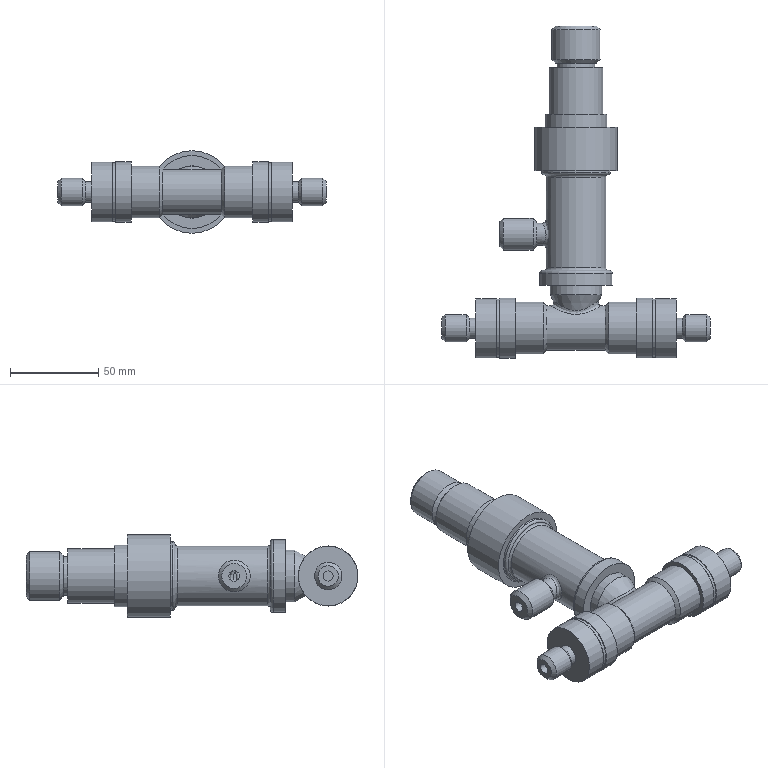Assembly | NX | mm | 17 component files | 17 solids | 192 faces | box 152 x 188.1 x 46.8 mm | volume 198339 mm3 | plane 85 | cylinder 66 | spline 22 | cone 15 | torus 4 | commonest cylinder face diameters 24 x4 16.6 x4 6 x3 29.4 x3 13 x3 17.4 x3 18 x3 33.8 x3
Bill of materials:
unnamed part 1 | 1 |  | Hollow cylindrical tube body with an enlarged collar at one end, a stepped larger-diameter band at the other end, and a short, smaller cylindrical side branch near the collar end; the side branch has a neck and a chamfered end.
unnamed part 2 | 1 |  | Tee-shaped hollow body: a straight cylindrical run with stepped, larger-diameter ends and a perpendicular branch that has a wider base section and a narrower cylindrical extension.
unnamed part 3 | 2 |  | Helical coil of round wire with open-pitch coils; at least one end coil appears flattened or ground to a flat ring face.
unnamed part 4 | 1 |  | Long helical coil of round wire with open pitch and flattened/closed end coils.
unnamed part 5 | 2 |  | Plain solid circular disc: a short cylinder with flat, parallel faces and no visible holes or features.
unnamed part 6 | 2 |  | Stepped axisymmetric body: a large cylinder, a wider flange-like collar, a narrow neck, and a smaller chamfered cylindrical tip with a small axial bore.
unnamed part 7 | 2 |  | Solid right circular cylinder (plug/slug shape) with flat ends and a length somewhat less than its diameter.
unnamed part 8 | 1 |  | Helical coil of round wire with open pitch and flat-faced end coils, similar in form to a compression spring.
unnamed part 9 | 2 |  | Thin flat annular ring (washer-like) with a large central hole and uniform rectangular cross-section.
unnamed part 10 | 1 |  | Short cylindrical disc/plug with chamfered edges on both faces and a hexagonal through-opening on the axis.
unnamed part 11 | 1 |  | Hollow cylindrical sleeve/tube with a round bore and plain cylindrical outer surface; length similar to diameter.
unnamed part 12 | 1 |  | Stepped axisymmetric body: a large hollow cup-like end, intermediate cylindrical steps, a narrow neck groove, and a smaller chamfered cylindrical tip with a small axial bore.
Mates:
1. fix | check_valve 1 component
2. concentric | valve_port 2 edge | washer 2 edge
3. concentric | washer 2 edge | check_valve 1 edge
4. concentric | valve_body 1 edge | check_valve 1 edge
5. concentric | spring_seat 1 edge | valve_body 1 edge
6. concentric | vent_valve 1 edge | valve_body 1 edge
7. touch align | adj_nut 1 face | vent_valve 1 face
8. distance | adj_nut 1 face | vent_valve 1 face
9. concentric | vent_spring 1 edge | spring_seat 1 edge
10. concentric | valve_port_filter 2 edge | valve_port 2 edge
11. concentric | valve_port_spring 2 edge | valve_port_filter 2 edge
12. concentric | washer 1 edge | check_valve 1 edge
13. concentric | valve_port 1 edge | washer 1 edge
14. concentric | valve_port_filter 1 edge | valve_port 1 edge
15. concentric | valve_port_spring 1 edge | valve_port_filter 1 edge
16. concentric | valve_body_filter 2 edge | check_valve 1 edge
17. concentric | valve_body_filter 1 edge | valve_body 1 edge
18. concentric | valve_body_spring 1 edge | valve_body_filter 2 edge